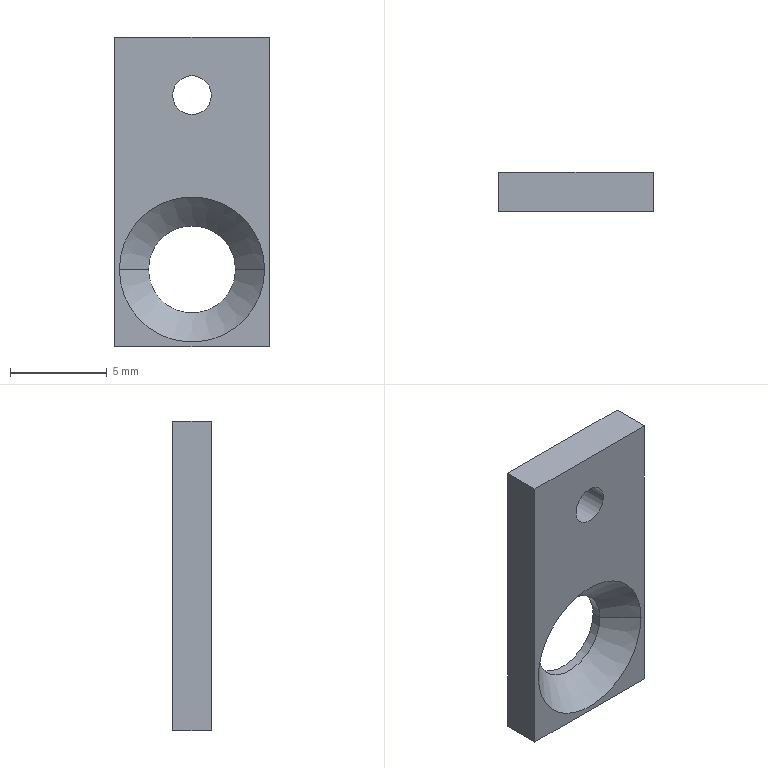Component | SolidWorks | BSH3-02-00ARubberBlankingAssembly2-1_BSH3-02-06SpringRetainer-1 | 1 solid | 12 faces | box 8 x 2 x 16 mm | volume 198 mm3 | plane 6 | cylinder 4 | cone 2 | commonest cylinder face diameters 4.5 x2 2 x2
build123d program:
from build123d import *

# Parameters (mm, degrees)
SKETCH1_W      = 8
SKETCH1_H      = 16
SKETCH1_R      = 1
SKETCH1_R_2    = 2.25
EXTRUDE1_DEPTH = 2
CHAMFER1_SIZE  = 1.5


with BuildPart() as part:
    # Sketch1 → Extrude1 (new body)
    with BuildSketch(Plane.XY):
        Rectangle(SKETCH1_W, SKETCH1_H)
        with Locations((0, -5)):
            Circle(SKETCH1_R, mode=Mode.SUBTRACT)
        with Locations((0, 4)):
            Circle(SKETCH1_R_2, mode=Mode.SUBTRACT)
    extrude(amount=EXTRUDE1_DEPTH)

    # Chamfer1
    chamfer1_edges = [part.edges().sort_by_distance(p)[0] for p in [
        (-2.25, 4, 2),
    ]]
    chamfer(chamfer1_edges, length=CHAMFER1_SIZE)


solid = part.part

# Placed as in the assembly
solid = solid.moved(Location((102.629, 14.262, -7.239), (90, 0, -180)))
STEP:
#1=COLOUR_RGB('',0.7922,0.8196,0.9333);
#2=FILL_AREA_STYLE_COLOUR('',#1);
#3=FILL_AREA_STYLE('',(#2));
#4=SURFACE_STYLE_FILL_AREA(#3);
#5=SURFACE_SIDE_STYLE('',(#4));
#6=SURFACE_STYLE_USAGE(.BOTH.,#5);
#7=PRESENTATION_STYLE_ASSIGNMENT((#6));
#8=CARTESIAN_POINT('',(4.129,0.5418,-0.4425));
#9=VERTEX_POINT('',#8);
#10=CARTESIAN_POINT('',(3.952,0.5418,-0.4425));
#11=VERTEX_POINT('',#10);
#12=CARTESIAN_POINT('',(4.041,0.5418,-0.4425));
#13=DIRECTION('',(0.,-1.,0.));
#14=DIRECTION('',(1.,0.,0.));
#15=AXIS2_PLACEMENT_3D('',#12,#13,#14);
#16=CIRCLE('',#15,0.08858);
#17=EDGE_CURVE('',#9,#11,#16,.T.);
#18=ORIENTED_EDGE('',*,*,#17,.F.);
#19=CARTESIAN_POINT('',(4.188,0.4827,-0.4425));
#20=VERTEX_POINT('',#19);
#21=CARTESIAN_POINT('',(4.129,0.5418,-0.4425));
#22=DIRECTION('',(0.7071,-0.7071,-0.));
#23=VECTOR('',#22,39.37);
#24=LINE('',#21,#23);
#25=EDGE_CURVE('',#9,#20,#24,.T.);
#26=ORIENTED_EDGE('',*,*,#25,.T.);
#27=CARTESIAN_POINT('',(3.893,0.4827,-0.4425));
#28=VERTEX_POINT('',#27);
#29=CARTESIAN_POINT('',(4.041,0.4827,-0.4425));
#30=DIRECTION('',(-0.,1.,-0.));
#31=DIRECTION('',(1.,0.,0.));
#32=AXIS2_PLACEMENT_3D('',#29,#30,#31);
#33=CIRCLE('',#32,0.1476);
#34=EDGE_CURVE('',#28,#20,#33,.T.);
#35=ORIENTED_EDGE('',*,*,#34,.F.);
#36=CARTESIAN_POINT('',(3.952,0.5418,-0.4425));
#37=DIRECTION('',(-0.7071,-0.7071,0.));
#38=VECTOR('',#37,39.37);
#39=LINE('',#36,#38);
#40=EDGE_CURVE('',#11,#28,#39,.T.);
#41=ORIENTED_EDGE('',*,*,#40,.F.);
#42=EDGE_LOOP('',(#18,#26,#35,#41));
#43=FACE_OUTER_BOUND('',#42,.T.);
#44=CARTESIAN_POINT('',(4.041,0.5418,-0.4425));
#45=DIRECTION('',(0.,-1.,0.));
#46=DIRECTION('',(-1.,0.,0.));
#47=AXIS2_PLACEMENT_3D('',#44,#45,#46);
#48=CONICAL_SURFACE('',#47,0.08858,0.7854);
#49=ADVANCED_FACE('',(#43),#48,.F.);
#50=ORIENTED_EDGE('',*,*,#17,.T.);
#51=CARTESIAN_POINT('',(3.952,0.5615,-0.4425));
#52=VERTEX_POINT('',#51);
#53=CARTESIAN_POINT('',(3.952,0.4827,-0.4425));
#54=DIRECTION('',(-0.,1.,-0.));
#55=VECTOR('',#54,39.37);
#56=LINE('',#53,#55);
#57=EDGE_CURVE('',#11,#52,#56,.T.);
#58=ORIENTED_EDGE('',*,*,#57,.T.);
#59=CARTESIAN_POINT('',(4.129,0.5615,-0.4425));
#60=VERTEX_POINT('',#59);
#61=CARTESIAN_POINT('',(4.041,0.5615,-0.4425));
#62=DIRECTION('',(0.,-1.,0.));
#63=DIRECTION('',(-1.,0.,0.));
#64=AXIS2_PLACEMENT_3D('',#61,#62,#63);
#65=CIRCLE('',#64,0.08858);
#66=EDGE_CURVE('',#60,#52,#65,.T.);
#67=ORIENTED_EDGE('',*,*,#66,.F.);
#68=CARTESIAN_POINT('',(4.129,0.4827,-0.4425));
#69=DIRECTION('',(-0.,1.,-0.));
#70=VECTOR('',#69,39.37);
#71=LINE('',#68,#70);
#72=EDGE_CURVE('',#9,#60,#71,.T.);
#73=ORIENTED_EDGE('',*,*,#72,.F.);
#74=EDGE_LOOP('',(#50,#58,#67,#73));
#75=FACE_OUTER_BOUND('',#74,.T.);
#76=CARTESIAN_POINT('',(4.041,0.4827,-0.4425));
#77=DIRECTION('',(-0.,1.,-0.));
#78=DIRECTION('',(1.,0.,0.));
#79=AXIS2_PLACEMENT_3D('',#76,#77,#78);
#80=CYLINDRICAL_SURFACE('',#79,0.08858);
#81=ADVANCED_FACE('',(#75),#80,.F.);
#82=CARTESIAN_POINT('',(4.08,0.4827,-0.08816));
#83=VERTEX_POINT('',#82);
#84=CARTESIAN_POINT('',(4.001,0.4827,-0.08816));
#85=VERTEX_POINT('',#84);
#86=CARTESIAN_POINT('',(4.041,0.4827,-0.08816));
#87=DIRECTION('',(0.,-1.,0.));
#88=DIRECTION('',(-1.,0.,0.));
#89=AXIS2_PLACEMENT_3D('',#86,#87,#88);
#90=CIRCLE('',#89,0.03937);
#91=EDGE_CURVE('',#83,#85,#90,.T.);
#92=ORIENTED_EDGE('',*,*,#91,.T.);
#93=CARTESIAN_POINT('',(4.001,0.5615,-0.08816));
#94=VERTEX_POINT('',#93);
#95=CARTESIAN_POINT('',(4.001,0.4827,-0.08816));
#96=DIRECTION('',(-0.,1.,-0.));
#97=VECTOR('',#96,39.37);
#98=LINE('',#95,#97);
#99=EDGE_CURVE('',#85,#94,#98,.T.);
#100=ORIENTED_EDGE('',*,*,#99,.T.);
#101=CARTESIAN_POINT('',(4.08,0.5615,-0.08816));
#102=VERTEX_POINT('',#101);
#103=CARTESIAN_POINT('',(4.041,0.5615,-0.08816));
#104=DIRECTION('',(0.,-1.,0.));
#105=DIRECTION('',(-1.,0.,0.));
#106=AXIS2_PLACEMENT_3D('',#103,#104,#105);
#107=CIRCLE('',#106,0.03937);
#108=EDGE_CURVE('',#102,#94,#107,.T.);
#109=ORIENTED_EDGE('',*,*,#108,.F.);
#110=CARTESIAN_POINT('',(4.08,0.4827,-0.08816));
#111=DIRECTION('',(-0.,1.,-0.));
#112=VECTOR('',#111,39.37);
#113=LINE('',#110,#112);
#114=EDGE_CURVE('',#83,#102,#113,.T.);
#115=ORIENTED_EDGE('',*,*,#114,.F.);
#116=EDGE_LOOP('',(#92,#100,#109,#115));
#117=FACE_OUTER_BOUND('',#116,.T.);
#118=CARTESIAN_POINT('',(4.041,0.4827,-0.08816));
#119=DIRECTION('',(-0.,1.,-0.));
#120=DIRECTION('',(1.,0.,0.));
#121=AXIS2_PLACEMENT_3D('',#118,#119,#120);
#122=CYLINDRICAL_SURFACE('',#121,0.03937);
#123=ADVANCED_FACE('',(#117),#122,.F.);
#124=ORIENTED_EDGE('',*,*,#34,.T.);
#125=CARTESIAN_POINT('',(4.041,0.4827,-0.4425));
#126=DIRECTION('',(-0.,1.,-0.));
#127=DIRECTION('',(1.,0.,0.));
#128=AXIS2_PLACEMENT_3D('',#125,#126,#127);
#129=CIRCLE('',#128,0.1476);
#130=EDGE_CURVE('',#20,#28,#129,.T.);
#131=ORIENTED_EDGE('',*,*,#130,.T.);
#132=EDGE_LOOP('',(#124,#131));
#133=FACE_BOUND('',#132,.T.);
#134=ORIENTED_EDGE('',*,*,#91,.F.);
#135=CARTESIAN_POINT('',(4.041,0.4827,-0.08816));
#136=DIRECTION('',(0.,-1.,0.));
#137=DIRECTION('',(-1.,0.,0.));
#138=AXIS2_PLACEMENT_3D('',#135,#136,#137);
#139=CIRCLE('',#138,0.03937);
#140=EDGE_CURVE('',#85,#83,#139,.T.);
#141=ORIENTED_EDGE('',*,*,#140,.F.);
#142=EDGE_LOOP('',(#134,#141));
#143=FACE_BOUND('',#142,.T.);
#144=CARTESIAN_POINT('',(3.883,0.4827,0.02995));
#145=VERTEX_POINT('',#144);
#146=CARTESIAN_POINT('',(3.883,0.4827,-0.6));
#147=VERTEX_POINT('',#146);
#148=CARTESIAN_POINT('',(3.883,0.4827,0.02995));
#149=DIRECTION('',(-0.,-0.,-1.));
#150=VECTOR('',#149,39.37);
#151=LINE('',#148,#150);
#152=EDGE_CURVE('',#145,#147,#151,.T.);
#153=ORIENTED_EDGE('',*,*,#152,.T.);
#154=CARTESIAN_POINT('',(4.198,0.4827,-0.6));
#155=VERTEX_POINT('',#154);
#156=CARTESIAN_POINT('',(4.198,0.4827,-0.6));
#157=DIRECTION('',(1.,0.,-0.));
#158=VECTOR('',#157,39.37);
#159=LINE('',#156,#158);
#160=EDGE_CURVE('',#147,#155,#159,.T.);
#161=ORIENTED_EDGE('',*,*,#160,.T.);
#162=CARTESIAN_POINT('',(4.198,0.4827,0.02995));
#163=VERTEX_POINT('',#162);
#164=CARTESIAN_POINT('',(4.198,0.4827,0.02995));
#165=DIRECTION('',(0.,0.,1.));
#166=VECTOR('',#165,39.37);
#167=LINE('',#164,#166);
#168=EDGE_CURVE('',#155,#163,#167,.T.);
#169=ORIENTED_EDGE('',*,*,#168,.T.);
#170=CARTESIAN_POINT('',(4.198,0.4827,0.02995));
#171=DIRECTION('',(-1.,-0.,0.));
#172=VECTOR('',#171,39.37);
#173=LINE('',#170,#172);
#174=EDGE_CURVE('',#163,#145,#173,.T.);
#175=ORIENTED_EDGE('',*,*,#174,.T.);
#176=EDGE_LOOP('',(#153,#161,#169,#175));
#177=FACE_OUTER_BOUND('',#176,.T.);
#178=CARTESIAN_POINT('',(3.883,0.4827,-0.6));
#179=DIRECTION('',(-0.,1.,-0.));
#180=DIRECTION('',(1.,0.,-0.));
#181=AXIS2_PLACEMENT_3D('',#178,#179,#180);
#182=PLANE('',#181);
#183=ADVANCED_FACE('',(#133,#143,#177),#182,.F.);
#184=ORIENTED_EDGE('',*,*,#108,.T.);
#185=CARTESIAN_POINT('',(4.041,0.5615,-0.08816));
#186=DIRECTION('',(0.,-1.,0.));
#187=DIRECTION('',(-1.,0.,0.));
#188=AXIS2_PLACEMENT_3D('',#185,#186,#187);
#189=CIRCLE('',#188,0.03937);
#190=EDGE_CURVE('',#94,#102,#189,.T.);
#191=ORIENTED_EDGE('',*,*,#190,.T.);
#192=EDGE_LOOP('',(#184,#191));
#193=FACE_BOUND('',#192,.T.);
#194=CARTESIAN_POINT('',(3.883,0.5615,0.02995));
#195=VERTEX_POINT('',#194);
#196=CARTESIAN_POINT('',(3.883,0.5615,-0.6));
#197=VERTEX_POINT('',#196);
#198=CARTESIAN_POINT('',(3.883,0.5615,0.02995));
#199=DIRECTION('',(-0.,-0.,-1.));
#200=VECTOR('',#199,39.37);
#201=LINE('',#198,#200);
#202=EDGE_CURVE('',#195,#197,#201,.T.);
#203=ORIENTED_EDGE('',*,*,#202,.F.);
#204=CARTESIAN_POINT('',(4.198,0.5615,0.02995));
#205=VERTEX_POINT('',#204);
#206=CARTESIAN_POINT('',(4.198,0.5615,0.02995));
#207=DIRECTION('',(-1.,-0.,0.));
#208=VECTOR('',#207,39.37);
#209=LINE('',#206,#208);
#210=EDGE_CURVE('',#205,#195,#209,.T.);
#211=ORIENTED_EDGE('',*,*,#210,.F.);
#212=CARTESIAN_POINT('',(4.198,0.5615,-0.6));
#213=VERTEX_POINT('',#212);
#214=CARTESIAN_POINT('',(4.198,0.5615,0.02995));
#215=DIRECTION('',(0.,0.,1.));
#216=VECTOR('',#215,39.37);
#217=LINE('',#214,#216);
#218=EDGE_CURVE('',#213,#205,#217,.T.);
#219=ORIENTED_EDGE('',*,*,#218,.F.);
#220=CARTESIAN_POINT('',(4.198,0.5615,-0.6));
#221=DIRECTION('',(1.,0.,-0.));
#222=VECTOR('',#221,39.37);
#223=LINE('',#220,#222);
#224=EDGE_CURVE('',#197,#213,#223,.T.);
#225=ORIENTED_EDGE('',*,*,#224,.F.);
#226=EDGE_LOOP('',(#203,#211,#219,#225));
#227=FACE_OUTER_BOUND('',#226,.T.);
#228=ORIENTED_EDGE('',*,*,#66,.T.);
#229=CARTESIAN_POINT('',(4.041,0.5615,-0.4425));
#230=DIRECTION('',(0.,-1.,0.));
#231=DIRECTION('',(-1.,0.,0.));
#232=AXIS2_PLACEMENT_3D('',#229,#230,#231);
#233=CIRCLE('',#232,0.08858);
#234=EDGE_CURVE('',#52,#60,#233,.T.);
#235=ORIENTED_EDGE('',*,*,#234,.T.);
#236=EDGE_LOOP('',(#228,#235));
#237=FACE_BOUND('',#236,.T.);
#238=CARTESIAN_POINT('',(3.883,0.5615,-0.6));
#239=DIRECTION('',(-0.,1.,-0.));
#240=DIRECTION('',(1.,0.,-0.));
#241=AXIS2_PLACEMENT_3D('',#238,#239,#240);
#242=PLANE('',#241);
#243=ADVANCED_FACE('',(#193,#227,#237),#242,.T.);
#244=ORIENTED_EDGE('',*,*,#202,.T.);
#245=CARTESIAN_POINT('',(3.883,0.4827,-0.6));
#246=DIRECTION('',(-0.,1.,-0.));
#247=VECTOR('',#246,39.37);
#248=LINE('',#245,#247);
#249=EDGE_CURVE('',#147,#197,#248,.T.);
#250=ORIENTED_EDGE('',*,*,#249,.F.);
#251=ORIENTED_EDGE('',*,*,#152,.F.);
#252=CARTESIAN_POINT('',(3.883,0.4827,0.02995));
#253=DIRECTION('',(-0.,1.,-0.));
#254=VECTOR('',#253,39.37);
#255=LINE('',#252,#254);
#256=EDGE_CURVE('',#145,#195,#255,.T.);
#257=ORIENTED_EDGE('',*,*,#256,.T.);
#258=EDGE_LOOP('',(#244,#250,#251,#257));
#259=FACE_OUTER_BOUND('',#258,.T.);
#260=CARTESIAN_POINT('',(3.883,0.4827,0.02995));
#261=DIRECTION('',(1.,0.,-0.));
#262=DIRECTION('',(0.,-1.,0.));
#263=AXIS2_PLACEMENT_3D('',#260,#261,#262);
#264=PLANE('',#263);
#265=ADVANCED_FACE('',(#259),#264,.F.);
#266=ORIENTED_EDGE('',*,*,#224,.T.);
#267=CARTESIAN_POINT('',(4.198,0.4827,-0.6));
#268=DIRECTION('',(-0.,1.,-0.));
#269=VECTOR('',#268,39.37);
#270=LINE('',#267,#269);
#271=EDGE_CURVE('',#155,#213,#270,.T.);
#272=ORIENTED_EDGE('',*,*,#271,.F.);
#273=ORIENTED_EDGE('',*,*,#160,.F.);
#274=ORIENTED_EDGE('',*,*,#249,.T.);
#275=EDGE_LOOP('',(#266,#272,#273,#274));
#276=FACE_OUTER_BOUND('',#275,.T.);
#277=CARTESIAN_POINT('',(4.198,0.4827,-0.6));
#278=DIRECTION('',(0.,0.,1.));
#279=DIRECTION('',(-0.,1.,-0.));
#280=AXIS2_PLACEMENT_3D('',#277,#278,#279);
#281=PLANE('',#280);
#282=ADVANCED_FACE('',(#276),#281,.F.);
#283=ORIENTED_EDGE('',*,*,#218,.T.);
#284=CARTESIAN_POINT('',(4.198,0.4827,0.02995));
#285=DIRECTION('',(-0.,1.,-0.));
#286=VECTOR('',#285,39.37);
#287=LINE('',#284,#286);
#288=EDGE_CURVE('',#163,#205,#287,.T.);
#289=ORIENTED_EDGE('',*,*,#288,.F.);
#290=ORIENTED_EDGE('',*,*,#168,.F.);
#291=ORIENTED_EDGE('',*,*,#271,.T.);
#292=EDGE_LOOP('',(#283,#289,#290,#291));
#293=FACE_OUTER_BOUND('',#292,.T.);
#294=CARTESIAN_POINT('',(4.198,0.4827,0.02995));
#295=DIRECTION('',(-1.,-0.,0.));
#296=DIRECTION('',(-0.,1.,-0.));
#297=AXIS2_PLACEMENT_3D('',#294,#295,#296);
#298=PLANE('',#297);
#299=ADVANCED_FACE('',(#293),#298,.F.);
#300=ORIENTED_EDGE('',*,*,#210,.T.);
#301=ORIENTED_EDGE('',*,*,#256,.F.);
#302=ORIENTED_EDGE('',*,*,#174,.F.);
#303=ORIENTED_EDGE('',*,*,#288,.T.);
#304=EDGE_LOOP('',(#300,#301,#302,#303));
#305=FACE_OUTER_BOUND('',#304,.T.);
#306=CARTESIAN_POINT('',(4.198,0.4827,0.02995));
#307=DIRECTION('',(-0.,-0.,-1.));
#308=DIRECTION('',(0.,-1.,0.));
#309=AXIS2_PLACEMENT_3D('',#306,#307,#308);
#310=PLANE('',#309);
#311=ADVANCED_FACE('',(#305),#310,.F.);
#312=ORIENTED_EDGE('',*,*,#99,.F.);
#313=ORIENTED_EDGE('',*,*,#140,.T.);
#314=ORIENTED_EDGE('',*,*,#114,.T.);
#315=ORIENTED_EDGE('',*,*,#190,.F.);
#316=EDGE_LOOP('',(#312,#313,#314,#315));
#317=FACE_OUTER_BOUND('',#316,.T.);
#318=CARTESIAN_POINT('',(4.041,0.4827,-0.08816));
#319=DIRECTION('',(-0.,1.,-0.));
#320=DIRECTION('',(1.,0.,0.));
#321=AXIS2_PLACEMENT_3D('',#318,#319,#320);
#322=CYLINDRICAL_SURFACE('',#321,0.03937);
#323=ADVANCED_FACE('',(#317),#322,.F.);
#324=ORIENTED_EDGE('',*,*,#57,.F.);
#325=CARTESIAN_POINT('',(4.041,0.5418,-0.4425));
#326=DIRECTION('',(0.,-1.,0.));
#327=DIRECTION('',(1.,0.,0.));
#328=AXIS2_PLACEMENT_3D('',#325,#326,#327);
#329=CIRCLE('',#328,0.08858);
#330=EDGE_CURVE('',#11,#9,#329,.T.);
#331=ORIENTED_EDGE('',*,*,#330,.T.);
#332=ORIENTED_EDGE('',*,*,#72,.T.);
#333=ORIENTED_EDGE('',*,*,#234,.F.);
#334=EDGE_LOOP('',(#324,#331,#332,#333));
#335=FACE_OUTER_BOUND('',#334,.T.);
#336=CARTESIAN_POINT('',(4.041,0.4827,-0.4425));
#337=DIRECTION('',(-0.,1.,-0.));
#338=DIRECTION('',(1.,0.,0.));
#339=AXIS2_PLACEMENT_3D('',#336,#337,#338);
#340=CYLINDRICAL_SURFACE('',#339,0.08858);
#341=ADVANCED_FACE('',(#335),#340,.F.);
#342=ORIENTED_EDGE('',*,*,#25,.F.);
#343=ORIENTED_EDGE('',*,*,#330,.F.);
#344=ORIENTED_EDGE('',*,*,#40,.T.);
#345=ORIENTED_EDGE('',*,*,#130,.F.);
#346=EDGE_LOOP('',(#342,#343,#344,#345));
#347=FACE_OUTER_BOUND('',#346,.T.);
#348=CARTESIAN_POINT('',(4.041,0.5418,-0.4425));
#349=DIRECTION('',(0.,-1.,0.));
#350=DIRECTION('',(-1.,0.,0.));
#351=AXIS2_PLACEMENT_3D('',#348,#349,#350);
#352=CONICAL_SURFACE('',#351,0.08858,0.7854);
#353=ADVANCED_FACE('',(#347),#352,.F.);
#354=CLOSED_SHELL('',(#49,#81,#123,#183,#243,#265,#282,#299,#311,#323,#341,#353));
#355=MANIFOLD_SOLID_BREP('',#354);
#356=STYLED_ITEM('',(#7),#355);
#357=PRESENTATION_LAYER_ASSIGNMENT('','',(#356));
#358=(LENGTH_UNIT()NAMED_UNIT(*)SI_UNIT($,.METRE.));
#359=LENGTH_MEASURE_WITH_UNIT(LENGTH_MEASURE(0.0254),#358);
#360=DIMENSIONAL_EXPONENTS(1.,0.,0.,0.,0.,0.,0.);
#361=(CONVERSION_BASED_UNIT('',#359)LENGTH_UNIT()NAMED_UNIT(#360));
#362=UNCERTAINTY_MEASURE_WITH_UNIT(LENGTH_MEASURE(0.00001),#361,'','');
#363=(NAMED_UNIT(*)PLANE_ANGLE_UNIT()SI_UNIT($,.RADIAN.));
#364=(NAMED_UNIT(*)SI_UNIT($,.STERADIAN.)SOLID_ANGLE_UNIT());
#365=(GEOMETRIC_REPRESENTATION_CONTEXT(3)GLOBAL_UNCERTAINTY_ASSIGNED_CONTEXT((#362))GLOBAL_UNIT_ASSIGNED_CONTEXT((#361,#363,#364))REPRESENTATION_CONTEXT('',''));
#366=MECHANICAL_DESIGN_GEOMETRIC_PRESENTATION_REPRESENTATION('',(#356),#365);
#367=CARTESIAN_POINT('',(0.,0.,0.));
#368=DIRECTION('',(0.,0.,1.));
#369=DIRECTION('',(1.,0.,0.));
#370=AXIS2_PLACEMENT_3D('',#367,#368,#369);
#371=(LENGTH_UNIT()NAMED_UNIT(*)SI_UNIT($,.METRE.));
#372=LENGTH_MEASURE_WITH_UNIT(LENGTH_MEASURE(0.0254),#371);
#373=DIMENSIONAL_EXPONENTS(1.,0.,0.,0.,0.,0.,0.);
#374=(CONVERSION_BASED_UNIT('',#372)LENGTH_UNIT()NAMED_UNIT(#373));
#375=UNCERTAINTY_MEASURE_WITH_UNIT(LENGTH_MEASURE(0.00001),#374,'','');
#376=(NAMED_UNIT(*)PLANE_ANGLE_UNIT()SI_UNIT($,.RADIAN.));
#377=(NAMED_UNIT(*)SI_UNIT($,.STERADIAN.)SOLID_ANGLE_UNIT());
#378=(GEOMETRIC_REPRESENTATION_CONTEXT(3)GLOBAL_UNCERTAINTY_ASSIGNED_CONTEXT((#375))GLOBAL_UNIT_ASSIGNED_CONTEXT((#374,#376,#377))REPRESENTATION_CONTEXT('',''));
#379=ADVANCED_BREP_SHAPE_REPRESENTATION('',(#355,#370),#378);